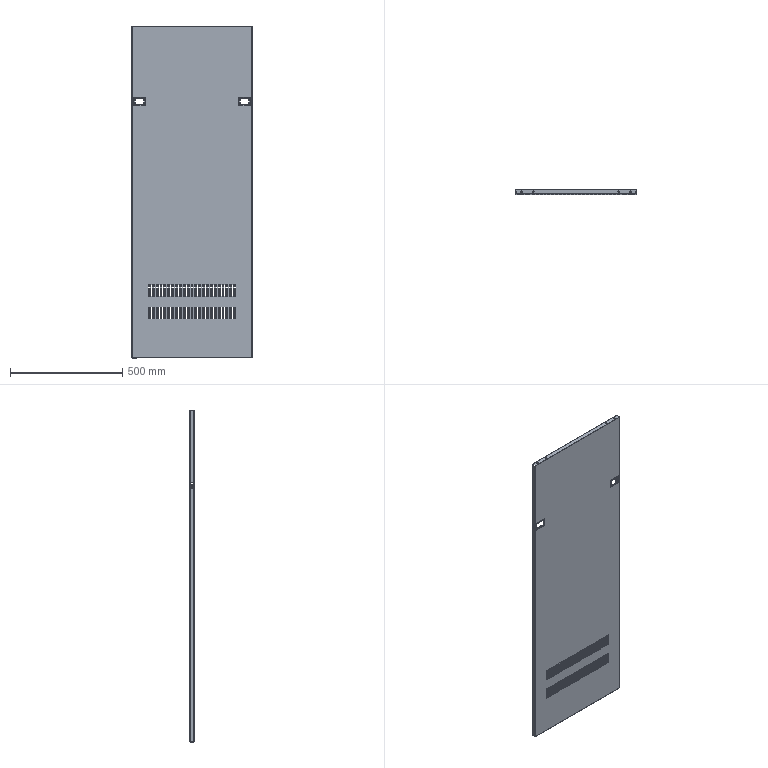Component | SolidWorks | RearDoorAssembly-1_RearDoor-1 | 1 solid | 386 faces | volume 1049582 mm3 | plane 338 | cylinder 32 | spline 16 | commonest cylinder face diameters 6.5 x16 0.2 x8 2.6 x8